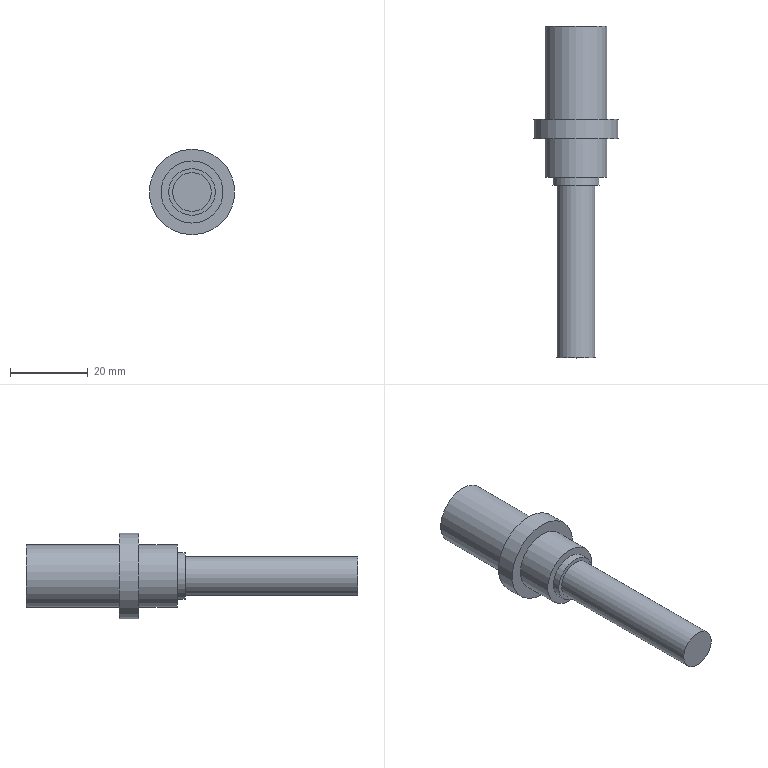Component | NX | DRIVE_SHAFT | 1 solid | 11 faces | box 22 x 85.5 x 22 mm | volume 12458 mm3 | plane 6 | cylinder 5 | commonest cylinder face diameters 16 x2 10 x1 12 x1 22 x1
STEP:
#1=CARTESIAN_POINT('',(0.,0.,0.));
#2=DIRECTION('',(0.,0.,1.));
#3=DIRECTION('',(1.,0.,0.));
#4=AXIS2_PLACEMENT_3D('',#1,#2,#3);
#5=CARTESIAN_POINT('',(-126.826,33.995,28.));
#6=VERTEX_POINT('',#5);
#7=CARTESIAN_POINT('',(-126.826,33.995,20.));
#8=DIRECTION('',(0.,-1.,0.));
#9=DIRECTION('',(0.,0.,1.));
#10=AXIS2_PLACEMENT_3D('',#7,#8,#9);
#11=CIRCLE('',#10,8.);
#12=CARTESIAN_POINT('',(-126.826,33.995,20.));
#13=DIRECTION('',(0.,-1.,0.));
#14=DIRECTION('',(0.,0.,1.));
#15=AXIS2_PLACEMENT_3D('',#12,#13,#14);
#16=PLANE('',#15);
#17=CARTESIAN_POINT('',(0.,0.));
#18=DIRECTION('',(1.,0.));
#19=AXIS2_PLACEMENT_2D('',#17,#18);
#20=CIRCLE('',#19,8.);
#21=(GEOMETRIC_REPRESENTATION_CONTEXT(2)PARAMETRIC_REPRESENTATION_CONTEXT()REPRESENTATION_CONTEXT('',''));
#22=DEFINITIONAL_REPRESENTATION('',(#20),#21);
#23=PCURVE('',#16,#22);
#24=CARTESIAN_POINT('',(-126.826,33.995,20.));
#25=DIRECTION('',(0.,-1.,0.));
#26=DIRECTION('',(0.,0.,1.));
#27=AXIS2_PLACEMENT_3D('',#24,#25,#26);
#28=CYLINDRICAL_SURFACE('',#27,8.);
#29=CARTESIAN_POINT('',(0.,0.));
#30=DIRECTION('',(1.,0.));
#31=VECTOR('',#30,1.);
#32=LINE('',#29,#31);
#33=(GEOMETRIC_REPRESENTATION_CONTEXT(2)PARAMETRIC_REPRESENTATION_CONTEXT()REPRESENTATION_CONTEXT('',''));
#34=DEFINITIONAL_REPRESENTATION('',(#32),#33);
#35=PCURVE('',#28,#34);
#36=SURFACE_CURVE('',#11,(#23,#35),.PCURVE_S1.);
#37=EDGE_CURVE('',#6,#6,#36,.T.);
#38=ORIENTED_EDGE('',*,*,#37,.F.);
#39=EDGE_LOOP('',(#38));
#40=FACE_BOUND('',#39,.T.);
#41=ADVANCED_FACE('',(#40),#16,.F.);
#42=CARTESIAN_POINT('',(-126.826,-51.505,25.));
#43=VERTEX_POINT('',#42);
#44=CARTESIAN_POINT('',(-126.826,-51.505,20.));
#45=DIRECTION('',(0.,-1.,0.));
#46=DIRECTION('',(0.,0.,1.));
#47=AXIS2_PLACEMENT_3D('',#44,#45,#46);
#48=CIRCLE('',#47,5.);
#49=CARTESIAN_POINT('',(-126.826,-51.505,20.));
#50=DIRECTION('',(0.,-1.,0.));
#51=DIRECTION('',(0.,0.,1.));
#52=AXIS2_PLACEMENT_3D('',#49,#50,#51);
#53=PLANE('',#52);
#54=CARTESIAN_POINT('',(0.,0.));
#55=DIRECTION('',(1.,0.));
#56=AXIS2_PLACEMENT_2D('',#54,#55);
#57=CIRCLE('',#56,5.);
#58=(GEOMETRIC_REPRESENTATION_CONTEXT(2)PARAMETRIC_REPRESENTATION_CONTEXT()REPRESENTATION_CONTEXT('',''));
#59=DEFINITIONAL_REPRESENTATION('',(#57),#58);
#60=PCURVE('',#53,#59);
#61=CARTESIAN_POINT('',(-126.826,33.995,20.));
#62=DIRECTION('',(0.,-1.,0.));
#63=DIRECTION('',(0.,0.,1.));
#64=AXIS2_PLACEMENT_3D('',#61,#62,#63);
#65=CYLINDRICAL_SURFACE('',#64,5.);
#66=CARTESIAN_POINT('',(0.,85.5));
#67=DIRECTION('',(1.,0.));
#68=VECTOR('',#67,1.);
#69=LINE('',#66,#68);
#70=(GEOMETRIC_REPRESENTATION_CONTEXT(2)PARAMETRIC_REPRESENTATION_CONTEXT()REPRESENTATION_CONTEXT('',''));
#71=DEFINITIONAL_REPRESENTATION('',(#69),#70);
#72=PCURVE('',#65,#71);
#73=SURFACE_CURVE('',#48,(#60,#72),.PCURVE_S1.);
#74=EDGE_CURVE('',#43,#43,#73,.T.);
#75=ORIENTED_EDGE('',*,*,#74,.T.);
#76=EDGE_LOOP('',(#75));
#77=FACE_BOUND('',#76,.T.);
#78=ADVANCED_FACE('',(#77),#53,.T.);
#79=ORIENTED_EDGE('',*,*,#74,.F.);
#80=CARTESIAN_POINT('',(-126.826,-7.005,25.));
#81=VERTEX_POINT('',#80);
#82=CARTESIAN_POINT('',(-126.826,-7.005,25.));
#83=CARTESIAN_POINT('',(-126.826,-51.505,25.));
#84=B_SPLINE_CURVE_WITH_KNOTS('',1,(#82,#83),.UNSPECIFIED.,.F.,.F.,(2,2),(41.,85.5),.PIECEWISE_BEZIER_KNOTS.);
#85=CARTESIAN_POINT('',(0.,0.));
#86=DIRECTION('',(0.,1.));
#87=VECTOR('',#86,1.);
#88=LINE('',#85,#87);
#89=(GEOMETRIC_REPRESENTATION_CONTEXT(2)PARAMETRIC_REPRESENTATION_CONTEXT()REPRESENTATION_CONTEXT('',''));
#90=DEFINITIONAL_REPRESENTATION('',(#88),#89);
#91=PCURVE('',#65,#90);
#92=CARTESIAN_POINT('',(6.283,0.));
#93=DIRECTION('',(0.,1.));
#94=VECTOR('',#93,1.);
#95=LINE('',#92,#94);
#96=(GEOMETRIC_REPRESENTATION_CONTEXT(2)PARAMETRIC_REPRESENTATION_CONTEXT()REPRESENTATION_CONTEXT('',''));
#97=DEFINITIONAL_REPRESENTATION('',(#95),#96);
#98=PCURVE('',#65,#97);
#99=SEAM_CURVE('',#84,(#91,#98),.PCURVE_S1.);
#100=EDGE_CURVE('',#81,#43,#99,.T.);
#101=ORIENTED_EDGE('',*,*,#100,.F.);
#102=CARTESIAN_POINT('',(-126.826,-7.005,15.));
#103=VERTEX_POINT('',#102);
#104=CARTESIAN_POINT('',(-126.826,-7.005,20.));
#105=DIRECTION('',(0.,-1.,0.));
#106=DIRECTION('',(0.,0.,-1.));
#107=AXIS2_PLACEMENT_3D('',#104,#105,#106);
#108=CIRCLE('',#107,5.);
#109=CARTESIAN_POINT('',(-3.142,41.));
#110=DIRECTION('',(1.,0.));
#111=VECTOR('',#110,1.);
#112=LINE('',#109,#111);
#113=(GEOMETRIC_REPRESENTATION_CONTEXT(2)PARAMETRIC_REPRESENTATION_CONTEXT()REPRESENTATION_CONTEXT('',''));
#114=DEFINITIONAL_REPRESENTATION('',(#112),#113);
#115=PCURVE('',#65,#114);
#116=CARTESIAN_POINT('',(-126.826,-7.005,26.));
#117=DIRECTION('',(0.,1.,0.));
#118=DIRECTION('',(0.,0.,-1.));
#119=AXIS2_PLACEMENT_3D('',#116,#117,#118);
#120=PLANE('',#119);
#121=CARTESIAN_POINT('',(11.,0.));
#122=CARTESIAN_POINT('',(11.,-8.66));
#123=CARTESIAN_POINT('',(3.5,-4.33));
#124=CARTESIAN_POINT('',(-4.,-0.));
#125=CARTESIAN_POINT('',(3.5,4.33));
#126=CARTESIAN_POINT('',(11.,8.66));
#127=CARTESIAN_POINT('',(11.,0.));
#128=(BOUNDED_CURVE()B_SPLINE_CURVE(2,(#121,#122,#123,#124,#125,#126,#127),.UNSPECIFIED.,.T.,.F.)B_SPLINE_CURVE_WITH_KNOTS((1,2,2,2,2,1),(-2.094,0.,2.094,4.189,6.283,8.378),.UNSPECIFIED.)CURVE()GEOMETRIC_REPRESENTATION_ITEM()RATIONAL_B_SPLINE_CURVE((1.,0.5,1.,0.5,1.,0.5,1.))REPRESENTATION_ITEM(''));
#129=(GEOMETRIC_REPRESENTATION_CONTEXT(2)PARAMETRIC_REPRESENTATION_CONTEXT()REPRESENTATION_CONTEXT('',''));
#130=DEFINITIONAL_REPRESENTATION('',(#128),#129);
#131=PCURVE('',#120,#130);
#132=SURFACE_CURVE('',#108,(#115,#131),.PCURVE_S1.);
#133=EDGE_CURVE('',#81,#103,#132,.T.);
#134=ORIENTED_EDGE('',*,*,#133,.T.);
#135=CARTESIAN_POINT('',(-126.826,-7.005,20.));
#136=DIRECTION('',(0.,-1.,0.));
#137=DIRECTION('',(0.,0.,-1.));
#138=AXIS2_PLACEMENT_3D('',#135,#136,#137);
#139=CIRCLE('',#138,5.);
#140=CARTESIAN_POINT('',(3.142,41.));
#141=DIRECTION('',(1.,0.));
#142=VECTOR('',#141,1.);
#143=LINE('',#140,#142);
#144=(GEOMETRIC_REPRESENTATION_CONTEXT(2)PARAMETRIC_REPRESENTATION_CONTEXT()REPRESENTATION_CONTEXT('',''));
#145=DEFINITIONAL_REPRESENTATION('',(#143),#144);
#146=PCURVE('',#65,#145);
#147=CARTESIAN_POINT('',(11.,0.));
#148=CARTESIAN_POINT('',(11.,-8.66));
#149=CARTESIAN_POINT('',(3.5,-4.33));
#150=CARTESIAN_POINT('',(-4.,-0.));
#151=CARTESIAN_POINT('',(3.5,4.33));
#152=CARTESIAN_POINT('',(11.,8.66));
#153=CARTESIAN_POINT('',(11.,0.));
#154=(BOUNDED_CURVE()B_SPLINE_CURVE(2,(#147,#148,#149,#150,#151,#152,#153),.UNSPECIFIED.,.T.,.F.)B_SPLINE_CURVE_WITH_KNOTS((1,2,2,2,2,1),(-2.094,0.,2.094,4.189,6.283,8.378),.UNSPECIFIED.)CURVE()GEOMETRIC_REPRESENTATION_ITEM()RATIONAL_B_SPLINE_CURVE((1.,0.5,1.,0.5,1.,0.5,1.))REPRESENTATION_ITEM(''));
#155=(GEOMETRIC_REPRESENTATION_CONTEXT(2)PARAMETRIC_REPRESENTATION_CONTEXT()REPRESENTATION_CONTEXT('',''));
#156=DEFINITIONAL_REPRESENTATION('',(#154),#155);
#157=PCURVE('',#120,#156);
#158=SURFACE_CURVE('',#139,(#146,#157),.PCURVE_S1.);
#159=EDGE_CURVE('',#103,#81,#158,.T.);
#160=ORIENTED_EDGE('',*,*,#159,.T.);
#161=ORIENTED_EDGE('',*,*,#100,.T.);
#162=EDGE_LOOP('',(#79,#101,#134,#160,#161));
#163=FACE_BOUND('',#162,.T.);
#164=ADVANCED_FACE('',(#163),#65,.T.);
#165=ORIENTED_EDGE('',*,*,#159,.F.);
#166=ORIENTED_EDGE('',*,*,#133,.F.);
#167=EDGE_LOOP('',(#165,#166));
#168=FACE_BOUND('',#167,.T.);
#169=CARTESIAN_POINT('',(-126.826,-7.005,14.));
#170=VERTEX_POINT('',#169);
#171=CARTESIAN_POINT('',(-126.826,-7.005,26.));
#172=VERTEX_POINT('',#171);
#173=CARTESIAN_POINT('',(-126.826,-7.005,20.));
#174=DIRECTION('',(0.,-1.,0.));
#175=DIRECTION('',(0.,0.,-1.));
#176=AXIS2_PLACEMENT_3D('',#173,#174,#175);
#177=CIRCLE('',#176,6.);
#178=CARTESIAN_POINT('',(12.,0.));
#179=CARTESIAN_POINT('',(12.,-10.392));
#180=CARTESIAN_POINT('',(3.,-5.196));
#181=CARTESIAN_POINT('',(-6.,-0.));
#182=CARTESIAN_POINT('',(3.,5.196));
#183=CARTESIAN_POINT('',(12.,10.392));
#184=CARTESIAN_POINT('',(12.,0.));
#185=(BOUNDED_CURVE()B_SPLINE_CURVE(2,(#178,#179,#180,#181,#182,#183,#184),.UNSPECIFIED.,.T.,.F.)B_SPLINE_CURVE_WITH_KNOTS((1,2,2,2,2,1),(-2.094,0.,2.094,4.189,6.283,8.378),.UNSPECIFIED.)CURVE()GEOMETRIC_REPRESENTATION_ITEM()RATIONAL_B_SPLINE_CURVE((1.,0.5,1.,0.5,1.,0.5,1.))REPRESENTATION_ITEM(''));
#186=(GEOMETRIC_REPRESENTATION_CONTEXT(2)PARAMETRIC_REPRESENTATION_CONTEXT()REPRESENTATION_CONTEXT('',''));
#187=DEFINITIONAL_REPRESENTATION('',(#185),#186);
#188=PCURVE('',#120,#187);
#189=CARTESIAN_POINT('',(-126.826,33.995,20.));
#190=DIRECTION('',(0.,-1.,0.));
#191=DIRECTION('',(0.,0.,1.));
#192=AXIS2_PLACEMENT_3D('',#189,#190,#191);
#193=CYLINDRICAL_SURFACE('',#192,6.);
#194=CARTESIAN_POINT('',(3.142,41.));
#195=DIRECTION('',(1.,0.));
#196=VECTOR('',#195,1.);
#197=LINE('',#194,#196);
#198=(GEOMETRIC_REPRESENTATION_CONTEXT(2)PARAMETRIC_REPRESENTATION_CONTEXT()REPRESENTATION_CONTEXT('',''));
#199=DEFINITIONAL_REPRESENTATION('',(#197),#198);
#200=PCURVE('',#193,#199);
#201=SURFACE_CURVE('',#177,(#188,#200),.PCURVE_S1.);
#202=EDGE_CURVE('',#170,#172,#201,.T.);
#203=ORIENTED_EDGE('',*,*,#202,.T.);
#204=CARTESIAN_POINT('',(-126.826,-7.005,20.));
#205=DIRECTION('',(0.,-1.,0.));
#206=DIRECTION('',(0.,0.,-1.));
#207=AXIS2_PLACEMENT_3D('',#204,#205,#206);
#208=CIRCLE('',#207,6.);
#209=CARTESIAN_POINT('',(12.,0.));
#210=CARTESIAN_POINT('',(12.,-10.392));
#211=CARTESIAN_POINT('',(3.,-5.196));
#212=CARTESIAN_POINT('',(-6.,-0.));
#213=CARTESIAN_POINT('',(3.,5.196));
#214=CARTESIAN_POINT('',(12.,10.392));
#215=CARTESIAN_POINT('',(12.,0.));
#216=(BOUNDED_CURVE()B_SPLINE_CURVE(2,(#209,#210,#211,#212,#213,#214,#215),.UNSPECIFIED.,.T.,.F.)B_SPLINE_CURVE_WITH_KNOTS((1,2,2,2,2,1),(-2.094,0.,2.094,4.189,6.283,8.378),.UNSPECIFIED.)CURVE()GEOMETRIC_REPRESENTATION_ITEM()RATIONAL_B_SPLINE_CURVE((1.,0.5,1.,0.5,1.,0.5,1.))REPRESENTATION_ITEM(''));
#217=(GEOMETRIC_REPRESENTATION_CONTEXT(2)PARAMETRIC_REPRESENTATION_CONTEXT()REPRESENTATION_CONTEXT('',''));
#218=DEFINITIONAL_REPRESENTATION('',(#216),#217);
#219=PCURVE('',#120,#218);
#220=CARTESIAN_POINT('',(-3.142,41.));
#221=DIRECTION('',(1.,0.));
#222=VECTOR('',#221,1.);
#223=LINE('',#220,#222);
#224=(GEOMETRIC_REPRESENTATION_CONTEXT(2)PARAMETRIC_REPRESENTATION_CONTEXT()REPRESENTATION_CONTEXT('',''));
#225=DEFINITIONAL_REPRESENTATION('',(#223),#224);
#226=PCURVE('',#193,#225);
#227=SURFACE_CURVE('',#208,(#219,#226),.PCURVE_S1.);
#228=EDGE_CURVE('',#172,#170,#227,.T.);
#229=ORIENTED_EDGE('',*,*,#228,.T.);
#230=EDGE_LOOP('',(#203,#229));
#231=FACE_BOUND('',#230,.T.);
#232=ADVANCED_FACE('',(#168,#231),#120,.F.);
#233=ORIENTED_EDGE('',*,*,#228,.F.);
#234=CARTESIAN_POINT('',(-126.826,-5.005,26.));
#235=VERTEX_POINT('',#234);
#236=CARTESIAN_POINT('',(-126.826,-5.005,26.));
#237=CARTESIAN_POINT('',(-126.826,-7.005,26.));
#238=B_SPLINE_CURVE_WITH_KNOTS('',1,(#236,#237),.UNSPECIFIED.,.F.,.F.,(2,2),(39.,41.),.PIECEWISE_BEZIER_KNOTS.);
#239=CARTESIAN_POINT('',(0.,0.));
#240=DIRECTION('',(0.,1.));
#241=VECTOR('',#240,1.);
#242=LINE('',#239,#241);
#243=(GEOMETRIC_REPRESENTATION_CONTEXT(2)PARAMETRIC_REPRESENTATION_CONTEXT()REPRESENTATION_CONTEXT('',''));
#244=DEFINITIONAL_REPRESENTATION('',(#242),#243);
#245=PCURVE('',#193,#244);
#246=CARTESIAN_POINT('',(6.283,0.));
#247=DIRECTION('',(0.,1.));
#248=VECTOR('',#247,1.);
#249=LINE('',#246,#248);
#250=(GEOMETRIC_REPRESENTATION_CONTEXT(2)PARAMETRIC_REPRESENTATION_CONTEXT()REPRESENTATION_CONTEXT('',''));
#251=DEFINITIONAL_REPRESENTATION('',(#249),#250);
#252=PCURVE('',#193,#251);
#253=SEAM_CURVE('',#238,(#245,#252),.PCURVE_S1.);
#254=EDGE_CURVE('',#235,#172,#253,.T.);
#255=ORIENTED_EDGE('',*,*,#254,.F.);
#256=CARTESIAN_POINT('',(-126.826,-5.005,20.));
#257=DIRECTION('',(0.,-1.,0.));
#258=DIRECTION('',(0.,0.,1.));
#259=AXIS2_PLACEMENT_3D('',#256,#257,#258);
#260=CIRCLE('',#259,6.);
#261=CARTESIAN_POINT('',(0.,39.));
#262=DIRECTION('',(1.,0.));
#263=VECTOR('',#262,1.);
#264=LINE('',#261,#263);
#265=(GEOMETRIC_REPRESENTATION_CONTEXT(2)PARAMETRIC_REPRESENTATION_CONTEXT()REPRESENTATION_CONTEXT('',''));
#266=DEFINITIONAL_REPRESENTATION('',(#264),#265);
#267=PCURVE('',#193,#266);
#268=CARTESIAN_POINT('',(-126.826,-5.005,28.));
#269=DIRECTION('',(0.,1.,0.));
#270=DIRECTION('',(0.,0.,-1.));
#271=AXIS2_PLACEMENT_3D('',#268,#269,#270);
#272=PLANE('',#271);
#273=CARTESIAN_POINT('',(2.,0.));
#274=CARTESIAN_POINT('',(2.,10.392));
#275=CARTESIAN_POINT('',(11.,5.196));
#276=CARTESIAN_POINT('',(20.,0.));
#277=CARTESIAN_POINT('',(11.,-5.196));
#278=CARTESIAN_POINT('',(2.,-10.392));
#279=CARTESIAN_POINT('',(2.,0.));
#280=(BOUNDED_CURVE()B_SPLINE_CURVE(2,(#273,#274,#275,#276,#277,#278,#279),.UNSPECIFIED.,.T.,.F.)B_SPLINE_CURVE_WITH_KNOTS((1,2,2,2,2,1),(-2.094,0.,2.094,4.189,6.283,8.378),.UNSPECIFIED.)CURVE()GEOMETRIC_REPRESENTATION_ITEM()RATIONAL_B_SPLINE_CURVE((1.,0.5,1.,0.5,1.,0.5,1.))REPRESENTATION_ITEM(''));
#281=(GEOMETRIC_REPRESENTATION_CONTEXT(2)PARAMETRIC_REPRESENTATION_CONTEXT()REPRESENTATION_CONTEXT('',''));
#282=DEFINITIONAL_REPRESENTATION('',(#280),#281);
#283=PCURVE('',#272,#282);
#284=SURFACE_CURVE('',#260,(#267,#283),.PCURVE_S1.);
#285=EDGE_CURVE('',#235,#235,#284,.T.);
#286=ORIENTED_EDGE('',*,*,#285,.T.);
#287=ORIENTED_EDGE('',*,*,#254,.T.);
#288=ORIENTED_EDGE('',*,*,#202,.F.);
#289=EDGE_LOOP('',(#233,#255,#286,#287,#288));
#290=FACE_BOUND('',#289,.T.);
#291=ADVANCED_FACE('',(#290),#193,.T.);
#292=ORIENTED_EDGE('',*,*,#285,.F.);
#293=EDGE_LOOP('',(#292));
#294=FACE_BOUND('',#293,.T.);
#295=CARTESIAN_POINT('',(-126.826,-5.005,28.));
#296=VERTEX_POINT('',#295);
#297=CARTESIAN_POINT('',(-126.826,-5.005,20.));
#298=DIRECTION('',(0.,-1.,0.));
#299=DIRECTION('',(0.,0.,1.));
#300=AXIS2_PLACEMENT_3D('',#297,#298,#299);
#301=CIRCLE('',#300,8.);
#302=CARTESIAN_POINT('',(0.,0.));
#303=CARTESIAN_POINT('',(0.,13.856));
#304=CARTESIAN_POINT('',(12.,6.928));
#305=CARTESIAN_POINT('',(24.,0.));
#306=CARTESIAN_POINT('',(12.,-6.928));
#307=CARTESIAN_POINT('',(0.,-13.856));
#308=CARTESIAN_POINT('',(0.,0.));
#309=(BOUNDED_CURVE()B_SPLINE_CURVE(2,(#302,#303,#304,#305,#306,#307,#308),.UNSPECIFIED.,.T.,.F.)B_SPLINE_CURVE_WITH_KNOTS((1,2,2,2,2,1),(-2.094,0.,2.094,4.189,6.283,8.378),.UNSPECIFIED.)CURVE()GEOMETRIC_REPRESENTATION_ITEM()RATIONAL_B_SPLINE_CURVE((1.,0.5,1.,0.5,1.,0.5,1.))REPRESENTATION_ITEM(''));
#310=(GEOMETRIC_REPRESENTATION_CONTEXT(2)PARAMETRIC_REPRESENTATION_CONTEXT()REPRESENTATION_CONTEXT('',''));
#311=DEFINITIONAL_REPRESENTATION('',(#309),#310);
#312=PCURVE('',#272,#311);
#313=CARTESIAN_POINT('',(-126.826,33.995,20.));
#314=DIRECTION('',(0.,-1.,0.));
#315=DIRECTION('',(0.,0.,1.));
#316=AXIS2_PLACEMENT_3D('',#313,#314,#315);
#317=CYLINDRICAL_SURFACE('',#316,8.);
#318=CARTESIAN_POINT('',(0.,39.));
#319=DIRECTION('',(1.,0.));
#320=VECTOR('',#319,1.);
#321=LINE('',#318,#320);
#322=(GEOMETRIC_REPRESENTATION_CONTEXT(2)PARAMETRIC_REPRESENTATION_CONTEXT()REPRESENTATION_CONTEXT('',''));
#323=DEFINITIONAL_REPRESENTATION('',(#321),#322);
#324=PCURVE('',#317,#323);
#325=SURFACE_CURVE('',#301,(#312,#324),.PCURVE_S1.);
#326=EDGE_CURVE('',#296,#296,#325,.T.);
#327=ORIENTED_EDGE('',*,*,#326,.T.);
#328=EDGE_LOOP('',(#327));
#329=FACE_BOUND('',#328,.T.);
#330=ADVANCED_FACE('',(#294,#329),#272,.F.);
#331=ORIENTED_EDGE('',*,*,#326,.F.);
#332=CARTESIAN_POINT('',(-126.826,4.995,28.));
#333=VERTEX_POINT('',#332);
#334=CARTESIAN_POINT('',(-126.826,4.995,28.));
#335=CARTESIAN_POINT('',(-126.826,-5.005,28.));
#336=B_SPLINE_CURVE_WITH_KNOTS('',1,(#334,#335),.UNSPECIFIED.,.F.,.F.,(2,2),(29.,39.),.PIECEWISE_BEZIER_KNOTS.);
#337=CARTESIAN_POINT('',(0.,0.));
#338=DIRECTION('',(0.,1.));
#339=VECTOR('',#338,1.);
#340=LINE('',#337,#339);
#341=(GEOMETRIC_REPRESENTATION_CONTEXT(2)PARAMETRIC_REPRESENTATION_CONTEXT()REPRESENTATION_CONTEXT('',''));
#342=DEFINITIONAL_REPRESENTATION('',(#340),#341);
#343=PCURVE('',#317,#342);
#344=CARTESIAN_POINT('',(6.283,0.));
#345=DIRECTION('',(0.,1.));
#346=VECTOR('',#345,1.);
#347=LINE('',#344,#346);
#348=(GEOMETRIC_REPRESENTATION_CONTEXT(2)PARAMETRIC_REPRESENTATION_CONTEXT()REPRESENTATION_CONTEXT('',''));
#349=DEFINITIONAL_REPRESENTATION('',(#347),#348);
#350=PCURVE('',#317,#349);
#351=SEAM_CURVE('',#336,(#343,#350),.PCURVE_S1.);
#352=EDGE_CURVE('',#333,#296,#351,.T.);
#353=ORIENTED_EDGE('',*,*,#352,.F.);
#354=CARTESIAN_POINT('',(-126.826,4.995,20.));
#355=DIRECTION('',(0.,-1.,0.));
#356=DIRECTION('',(0.,0.,1.));
#357=AXIS2_PLACEMENT_3D('',#354,#355,#356);
#358=CIRCLE('',#357,8.);
#359=CARTESIAN_POINT('',(0.,29.));
#360=DIRECTION('',(1.,0.));
#361=VECTOR('',#360,1.);
#362=LINE('',#359,#361);
#363=(GEOMETRIC_REPRESENTATION_CONTEXT(2)PARAMETRIC_REPRESENTATION_CONTEXT()REPRESENTATION_CONTEXT('',''));
#364=DEFINITIONAL_REPRESENTATION('',(#362),#363);
#365=PCURVE('',#317,#364);
#366=CARTESIAN_POINT('',(-126.826,4.995,31.));
#367=DIRECTION('',(0.,1.,0.));
#368=DIRECTION('',(0.,0.,-1.));
#369=AXIS2_PLACEMENT_3D('',#366,#367,#368);
#370=PLANE('',#369);
#371=CARTESIAN_POINT('',(3.,0.));
#372=CARTESIAN_POINT('',(3.,13.856));
#373=CARTESIAN_POINT('',(15.,6.928));
#374=CARTESIAN_POINT('',(27.,0.));
#375=CARTESIAN_POINT('',(15.,-6.928));
#376=CARTESIAN_POINT('',(3.,-13.856));
#377=CARTESIAN_POINT('',(3.,0.));
#378=(BOUNDED_CURVE()B_SPLINE_CURVE(2,(#371,#372,#373,#374,#375,#376,#377),.UNSPECIFIED.,.T.,.F.)B_SPLINE_CURVE_WITH_KNOTS((1,2,2,2,2,1),(-2.094,0.,2.094,4.189,6.283,8.378),.UNSPECIFIED.)CURVE()GEOMETRIC_REPRESENTATION_ITEM()RATIONAL_B_SPLINE_CURVE((1.,0.5,1.,0.5,1.,0.5,1.))REPRESENTATION_ITEM(''));
#379=(GEOMETRIC_REPRESENTATION_CONTEXT(2)PARAMETRIC_REPRESENTATION_CONTEXT()REPRESENTATION_CONTEXT('',''));
#380=DEFINITIONAL_REPRESENTATION('',(#378),#379);
#381=PCURVE('',#370,#380);
#382=SURFACE_CURVE('',#358,(#365,#381),.PCURVE_S1.);
#383=EDGE_CURVE('',#333,#333,#382,.T.);
#384=ORIENTED_EDGE('',*,*,#383,.T.);
#385=ORIENTED_EDGE('',*,*,#352,.T.);
#386=EDGE_LOOP('',(#331,#353,#384,#385));
#387=FACE_BOUND('',#386,.T.);
#388=ADVANCED_FACE('',(#387),#317,.T.);
#389=ORIENTED_EDGE('',*,*,#383,.F.);
#390=EDGE_LOOP('',(#389));
#391=FACE_BOUND('',#390,.T.);
#392=CARTESIAN_POINT('',(-126.826,4.995,31.));
#393=VERTEX_POINT('',#392);
#394=CARTESIAN_POINT('',(-126.826,4.995,20.));
#395=DIRECTION('',(0.,-1.,0.));
#396=DIRECTION('',(0.,0.,1.));
#397=AXIS2_PLACEMENT_3D('',#394,#395,#396);
#398=CIRCLE('',#397,11.);
#399=CARTESIAN_POINT('',(0.,0.));
#400=CARTESIAN_POINT('',(0.,19.053));
#401=CARTESIAN_POINT('',(16.5,9.526));
#402=CARTESIAN_POINT('',(33.,0.));
#403=CARTESIAN_POINT('',(16.5,-9.526));
#404=CARTESIAN_POINT('',(0.,-19.053));
#405=CARTESIAN_POINT('',(0.,0.));
#406=(BOUNDED_CURVE()B_SPLINE_CURVE(2,(#399,#400,#401,#402,#403,#404,#405),.UNSPECIFIED.,.T.,.F.)B_SPLINE_CURVE_WITH_KNOTS((1,2,2,2,2,1),(-2.094,0.,2.094,4.189,6.283,8.378),.UNSPECIFIED.)CURVE()GEOMETRIC_REPRESENTATION_ITEM()RATIONAL_B_SPLINE_CURVE((1.,0.5,1.,0.5,1.,0.5,1.))REPRESENTATION_ITEM(''));
#407=(GEOMETRIC_REPRESENTATION_CONTEXT(2)PARAMETRIC_REPRESENTATION_CONTEXT()REPRESENTATION_CONTEXT('',''));
#408=DEFINITIONAL_REPRESENTATION('',(#406),#407);
#409=PCURVE('',#370,#408);
#410=CARTESIAN_POINT('',(-126.826,33.995,20.));
#411=DIRECTION('',(0.,-1.,0.));
#412=DIRECTION('',(0.,0.,1.));
#413=AXIS2_PLACEMENT_3D('',#410,#411,#412);
#414=CYLINDRICAL_SURFACE('',#413,11.);
#415=CARTESIAN_POINT('',(0.,29.));
#416=DIRECTION('',(1.,0.));
#417=VECTOR('',#416,1.);
#418=LINE('',#415,#417);
#419=(GEOMETRIC_REPRESENTATION_CONTEXT(2)PARAMETRIC_REPRESENTATION_CONTEXT()REPRESENTATION_CONTEXT('',''));
#420=DEFINITIONAL_REPRESENTATION('',(#418),#419);
#421=PCURVE('',#414,#420);
#422=SURFACE_CURVE('',#398,(#409,#421),.PCURVE_S1.);
#423=EDGE_CURVE('',#393,#393,#422,.T.);
#424=ORIENTED_EDGE('',*,*,#423,.T.);
#425=EDGE_LOOP('',(#424));
#426=FACE_BOUND('',#425,.T.);
#427=ADVANCED_FACE('',(#391,#426),#370,.F.);
#428=ORIENTED_EDGE('',*,*,#423,.F.);
#429=CARTESIAN_POINT('',(-126.826,9.995,31.));
#430=VERTEX_POINT('',#429);
#431=CARTESIAN_POINT('',(-126.826,9.995,31.));
#432=CARTESIAN_POINT('',(-126.826,4.995,31.));
#433=B_SPLINE_CURVE_WITH_KNOTS('',1,(#431,#432),.UNSPECIFIED.,.F.,.F.,(2,2),(24.,29.),.PIECEWISE_BEZIER_KNOTS.);
#434=CARTESIAN_POINT('',(0.,0.));
#435=DIRECTION('',(0.,1.));
#436=VECTOR('',#435,1.);
#437=LINE('',#434,#436);
#438=(GEOMETRIC_REPRESENTATION_CONTEXT(2)PARAMETRIC_REPRESENTATION_CONTEXT()REPRESENTATION_CONTEXT('',''));
#439=DEFINITIONAL_REPRESENTATION('',(#437),#438);
#440=PCURVE('',#414,#439);
#441=CARTESIAN_POINT('',(6.283,0.));
#442=DIRECTION('',(0.,1.));
#443=VECTOR('',#442,1.);
#444=LINE('',#441,#443);
#445=(GEOMETRIC_REPRESENTATION_CONTEXT(2)PARAMETRIC_REPRESENTATION_CONTEXT()REPRESENTATION_CONTEXT('',''));
#446=DEFINITIONAL_REPRESENTATION('',(#444),#445);
#447=PCURVE('',#414,#446);
#448=SEAM_CURVE('',#433,(#440,#447),.PCURVE_S1.);
#449=EDGE_CURVE('',#430,#393,#448,.T.);
#450=ORIENTED_EDGE('',*,*,#449,.F.);
#451=CARTESIAN_POINT('',(-126.826,9.995,20.));
#452=DIRECTION('',(0.,-1.,0.));
#453=DIRECTION('',(0.,0.,1.));
#454=AXIS2_PLACEMENT_3D('',#451,#452,#453);
#455=CIRCLE('',#454,11.);
#456=CARTESIAN_POINT('',(0.,24.));
#457=DIRECTION('',(1.,0.));
#458=VECTOR('',#457,1.);
#459=LINE('',#456,#458);
#460=(GEOMETRIC_REPRESENTATION_CONTEXT(2)PARAMETRIC_REPRESENTATION_CONTEXT()REPRESENTATION_CONTEXT('',''));
#461=DEFINITIONAL_REPRESENTATION('',(#459),#460);
#462=PCURVE('',#414,#461);
#463=CARTESIAN_POINT('',(-126.826,9.995,28.));
#464=DIRECTION('',(0.,-1.,0.));
#465=DIRECTION('',(0.,0.,1.));
#466=AXIS2_PLACEMENT_3D('',#463,#464,#465);
#467=PLANE('',#466);
#468=CARTESIAN_POINT('',(-8.,0.));
#469=DIRECTION('',(1.,0.));
#470=AXIS2_PLACEMENT_2D('',#468,#469);
#471=CIRCLE('',#470,11.);
#472=(GEOMETRIC_REPRESENTATION_CONTEXT(2)PARAMETRIC_REPRESENTATION_CONTEXT()REPRESENTATION_CONTEXT('',''));
#473=DEFINITIONAL_REPRESENTATION('',(#471),#472);
#474=PCURVE('',#467,#473);
#475=SURFACE_CURVE('',#455,(#462,#474),.PCURVE_S1.);
#476=EDGE_CURVE('',#430,#430,#475,.T.);
#477=ORIENTED_EDGE('',*,*,#476,.T.);
#478=ORIENTED_EDGE('',*,*,#449,.T.);
#479=EDGE_LOOP('',(#428,#450,#477,#478));
#480=FACE_BOUND('',#479,.T.);
#481=ADVANCED_FACE('',(#480),#414,.T.);
#482=ORIENTED_EDGE('',*,*,#476,.F.);
#483=EDGE_LOOP('',(#482));
#484=FACE_BOUND('',#483,.T.);
#485=CARTESIAN_POINT('',(-126.826,9.995,28.));
#486=VERTEX_POINT('',#485);
#487=CARTESIAN_POINT('',(-126.826,9.995,20.));
#488=DIRECTION('',(0.,-1.,0.));
#489=DIRECTION('',(0.,0.,1.));
#490=AXIS2_PLACEMENT_3D('',#487,#488,#489);
#491=CIRCLE('',#490,8.);
#492=CARTESIAN_POINT('',(-8.,0.));
#493=DIRECTION('',(1.,0.));
#494=AXIS2_PLACEMENT_2D('',#492,#493);
#495=CIRCLE('',#494,8.);
#496=(GEOMETRIC_REPRESENTATION_CONTEXT(2)PARAMETRIC_REPRESENTATION_CONTEXT()REPRESENTATION_CONTEXT('',''));
#497=DEFINITIONAL_REPRESENTATION('',(#495),#496);
#498=PCURVE('',#467,#497);
#499=CARTESIAN_POINT('',(0.,24.));
#500=DIRECTION('',(1.,0.));
#501=VECTOR('',#500,1.);
#502=LINE('',#499,#501);
#503=(GEOMETRIC_REPRESENTATION_CONTEXT(2)PARAMETRIC_REPRESENTATION_CONTEXT()REPRESENTATION_CONTEXT('',''));
#504=DEFINITIONAL_REPRESENTATION('',(#502),#503);
#505=PCURVE('',#28,#504);
#506=SURFACE_CURVE('',#491,(#498,#505),.PCURVE_S1.);
#507=EDGE_CURVE('',#486,#486,#506,.T.);
#508=ORIENTED_EDGE('',*,*,#507,.T.);
#509=EDGE_LOOP('',(#508));
#510=FACE_BOUND('',#509,.T.);
#511=ADVANCED_FACE('',(#484,#510),#467,.F.);
#512=ORIENTED_EDGE('',*,*,#507,.F.);
#513=CARTESIAN_POINT('',(-126.826,33.995,28.));
#514=CARTESIAN_POINT('',(-126.826,9.995,28.));
#515=B_SPLINE_CURVE_WITH_KNOTS('',1,(#513,#514),.UNSPECIFIED.,.F.,.F.,(2,2),(0.,24.),.PIECEWISE_BEZIER_KNOTS.);
#516=CARTESIAN_POINT('',(0.,0.));
#517=DIRECTION('',(0.,1.));
#518=VECTOR('',#517,1.);
#519=LINE('',#516,#518);
#520=(GEOMETRIC_REPRESENTATION_CONTEXT(2)PARAMETRIC_REPRESENTATION_CONTEXT()REPRESENTATION_CONTEXT('',''));
#521=DEFINITIONAL_REPRESENTATION('',(#519),#520);
#522=PCURVE('',#28,#521);
#523=CARTESIAN_POINT('',(6.283,0.));
#524=DIRECTION('',(0.,1.));
#525=VECTOR('',#524,1.);
#526=LINE('',#523,#525);
#527=(GEOMETRIC_REPRESENTATION_CONTEXT(2)PARAMETRIC_REPRESENTATION_CONTEXT()REPRESENTATION_CONTEXT('',''));
#528=DEFINITIONAL_REPRESENTATION('',(#526),#527);
#529=PCURVE('',#28,#528);
#530=SEAM_CURVE('',#515,(#522,#529),.PCURVE_S1.);
#531=EDGE_CURVE('',#6,#486,#530,.T.);
#532=ORIENTED_EDGE('',*,*,#531,.F.);
#533=ORIENTED_EDGE('',*,*,#37,.T.);
#534=ORIENTED_EDGE('',*,*,#531,.T.);
#535=EDGE_LOOP('',(#512,#532,#533,#534));
#536=FACE_BOUND('',#535,.T.);
#537=ADVANCED_FACE('',(#536),#28,.T.);
#538=CLOSED_SHELL('',(#41,#78,#164,#232,#291,#330,#388,#427,#481,#511,#537));
#539=MANIFOLD_SOLID_BREP('',#538);
#540=(LENGTH_UNIT()NAMED_UNIT(*)SI_UNIT(.MILLI.,.METRE.));
#541=UNCERTAINTY_MEASURE_WITH_UNIT(LENGTH_MEASURE(0.000005),#540,'','');
#542=(NAMED_UNIT(*)PLANE_ANGLE_UNIT()SI_UNIT($,.RADIAN.));
#543=(NAMED_UNIT(*)SI_UNIT($,.STERADIAN.)SOLID_ANGLE_UNIT());
#544=(GEOMETRIC_REPRESENTATION_CONTEXT(3)GLOBAL_UNCERTAINTY_ASSIGNED_CONTEXT((#541))GLOBAL_UNIT_ASSIGNED_CONTEXT((#540,#542,#543))REPRESENTATION_CONTEXT('',''));
#545=ADVANCED_BREP_SHAPE_REPRESENTATION('',(#4,#539),#544);